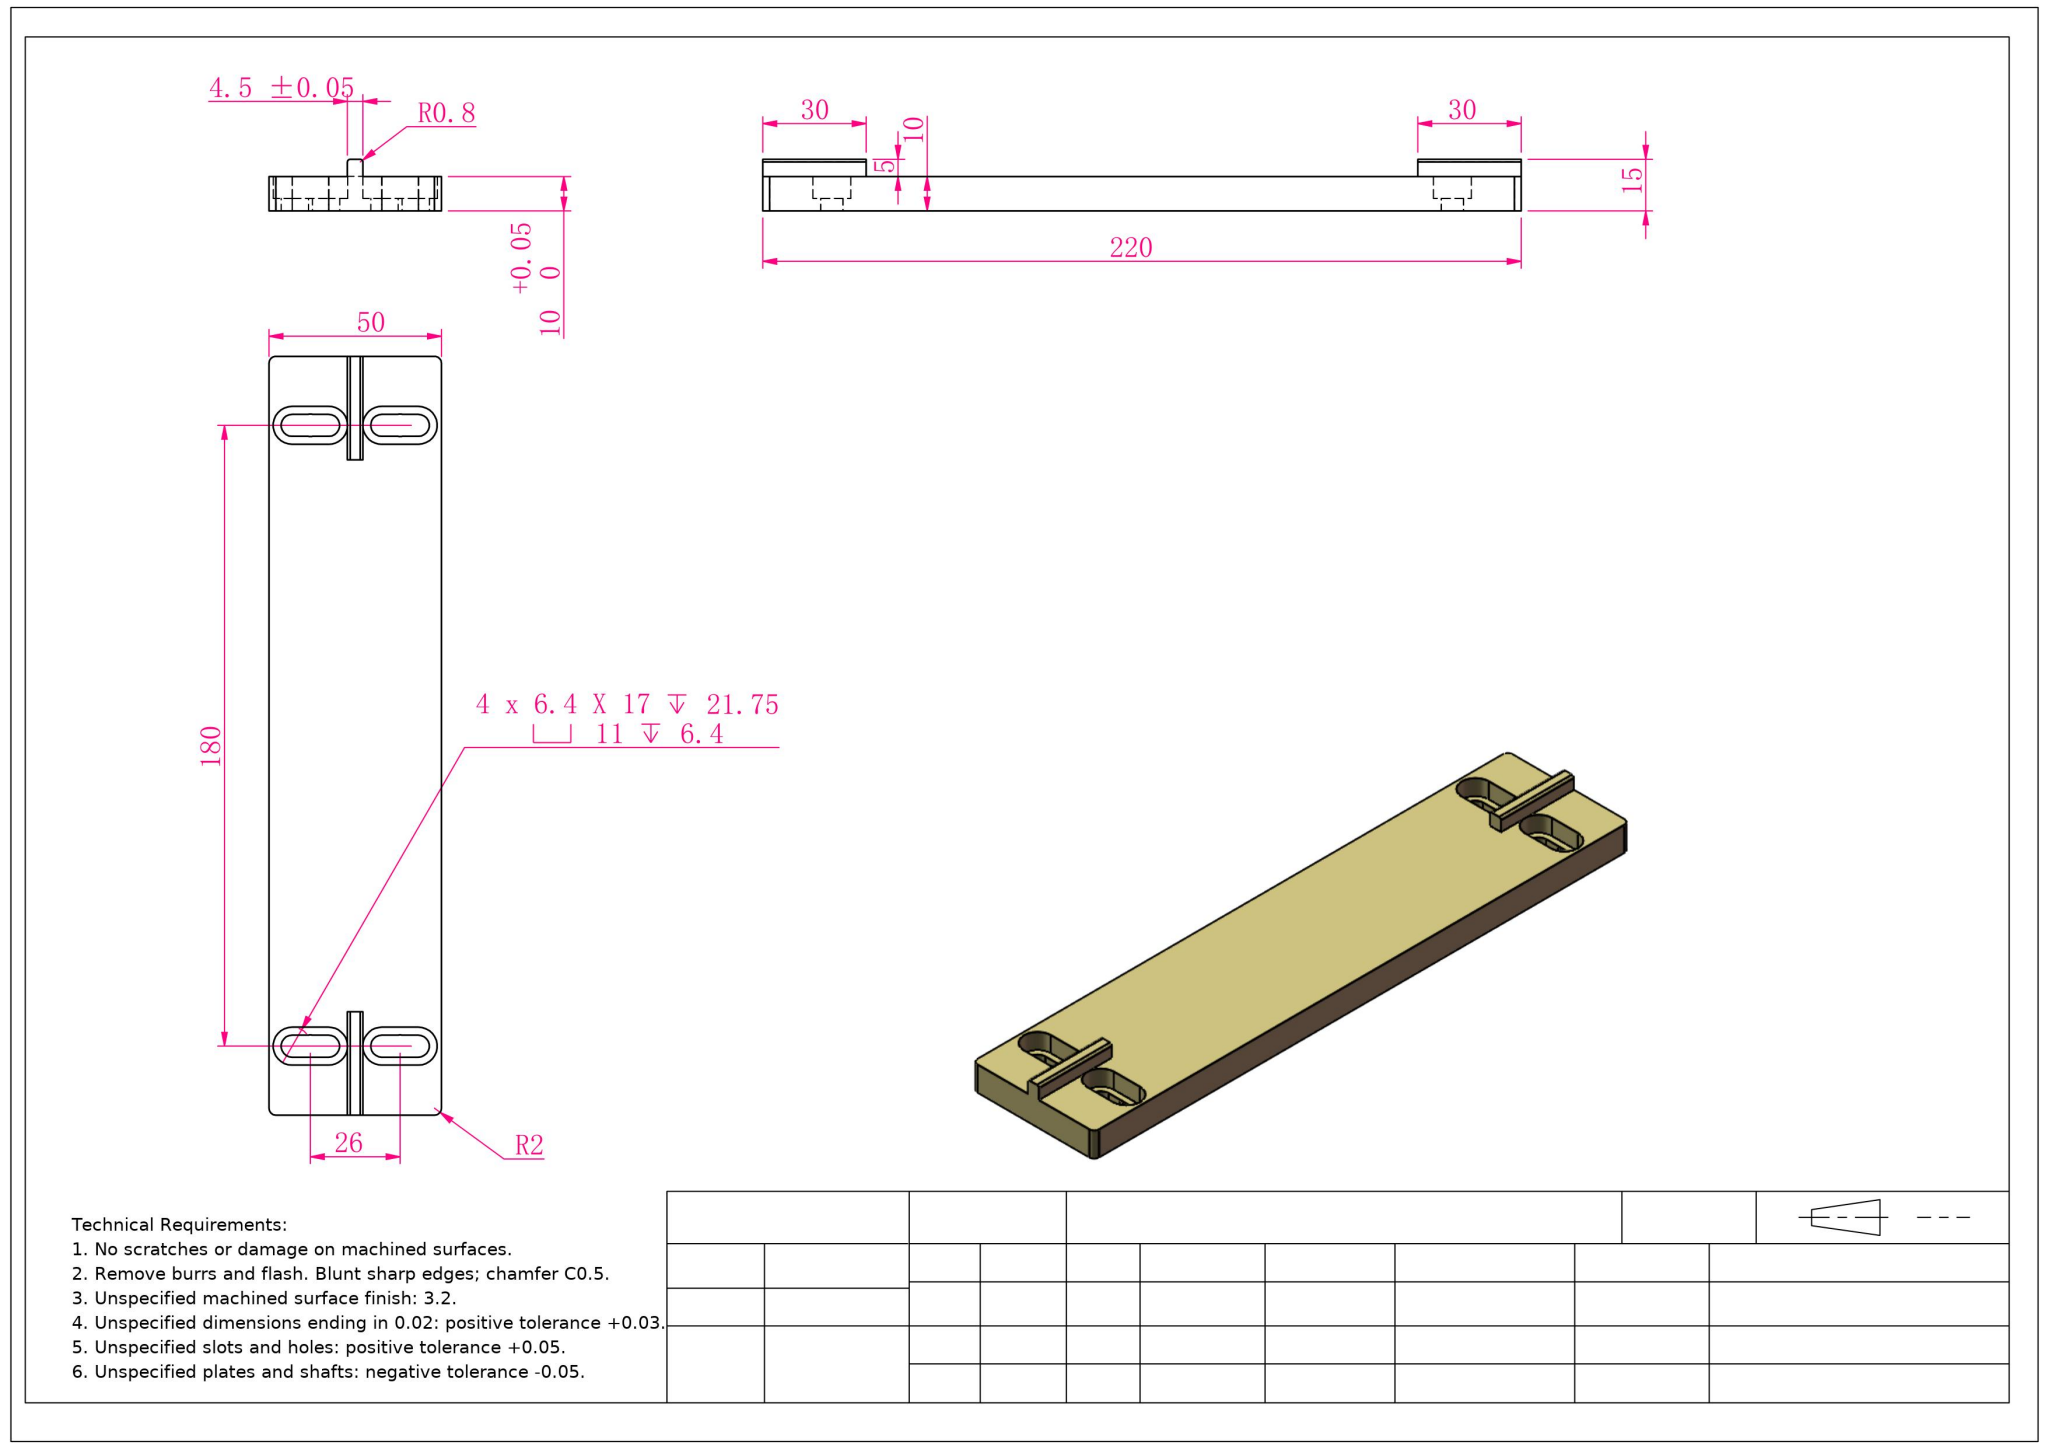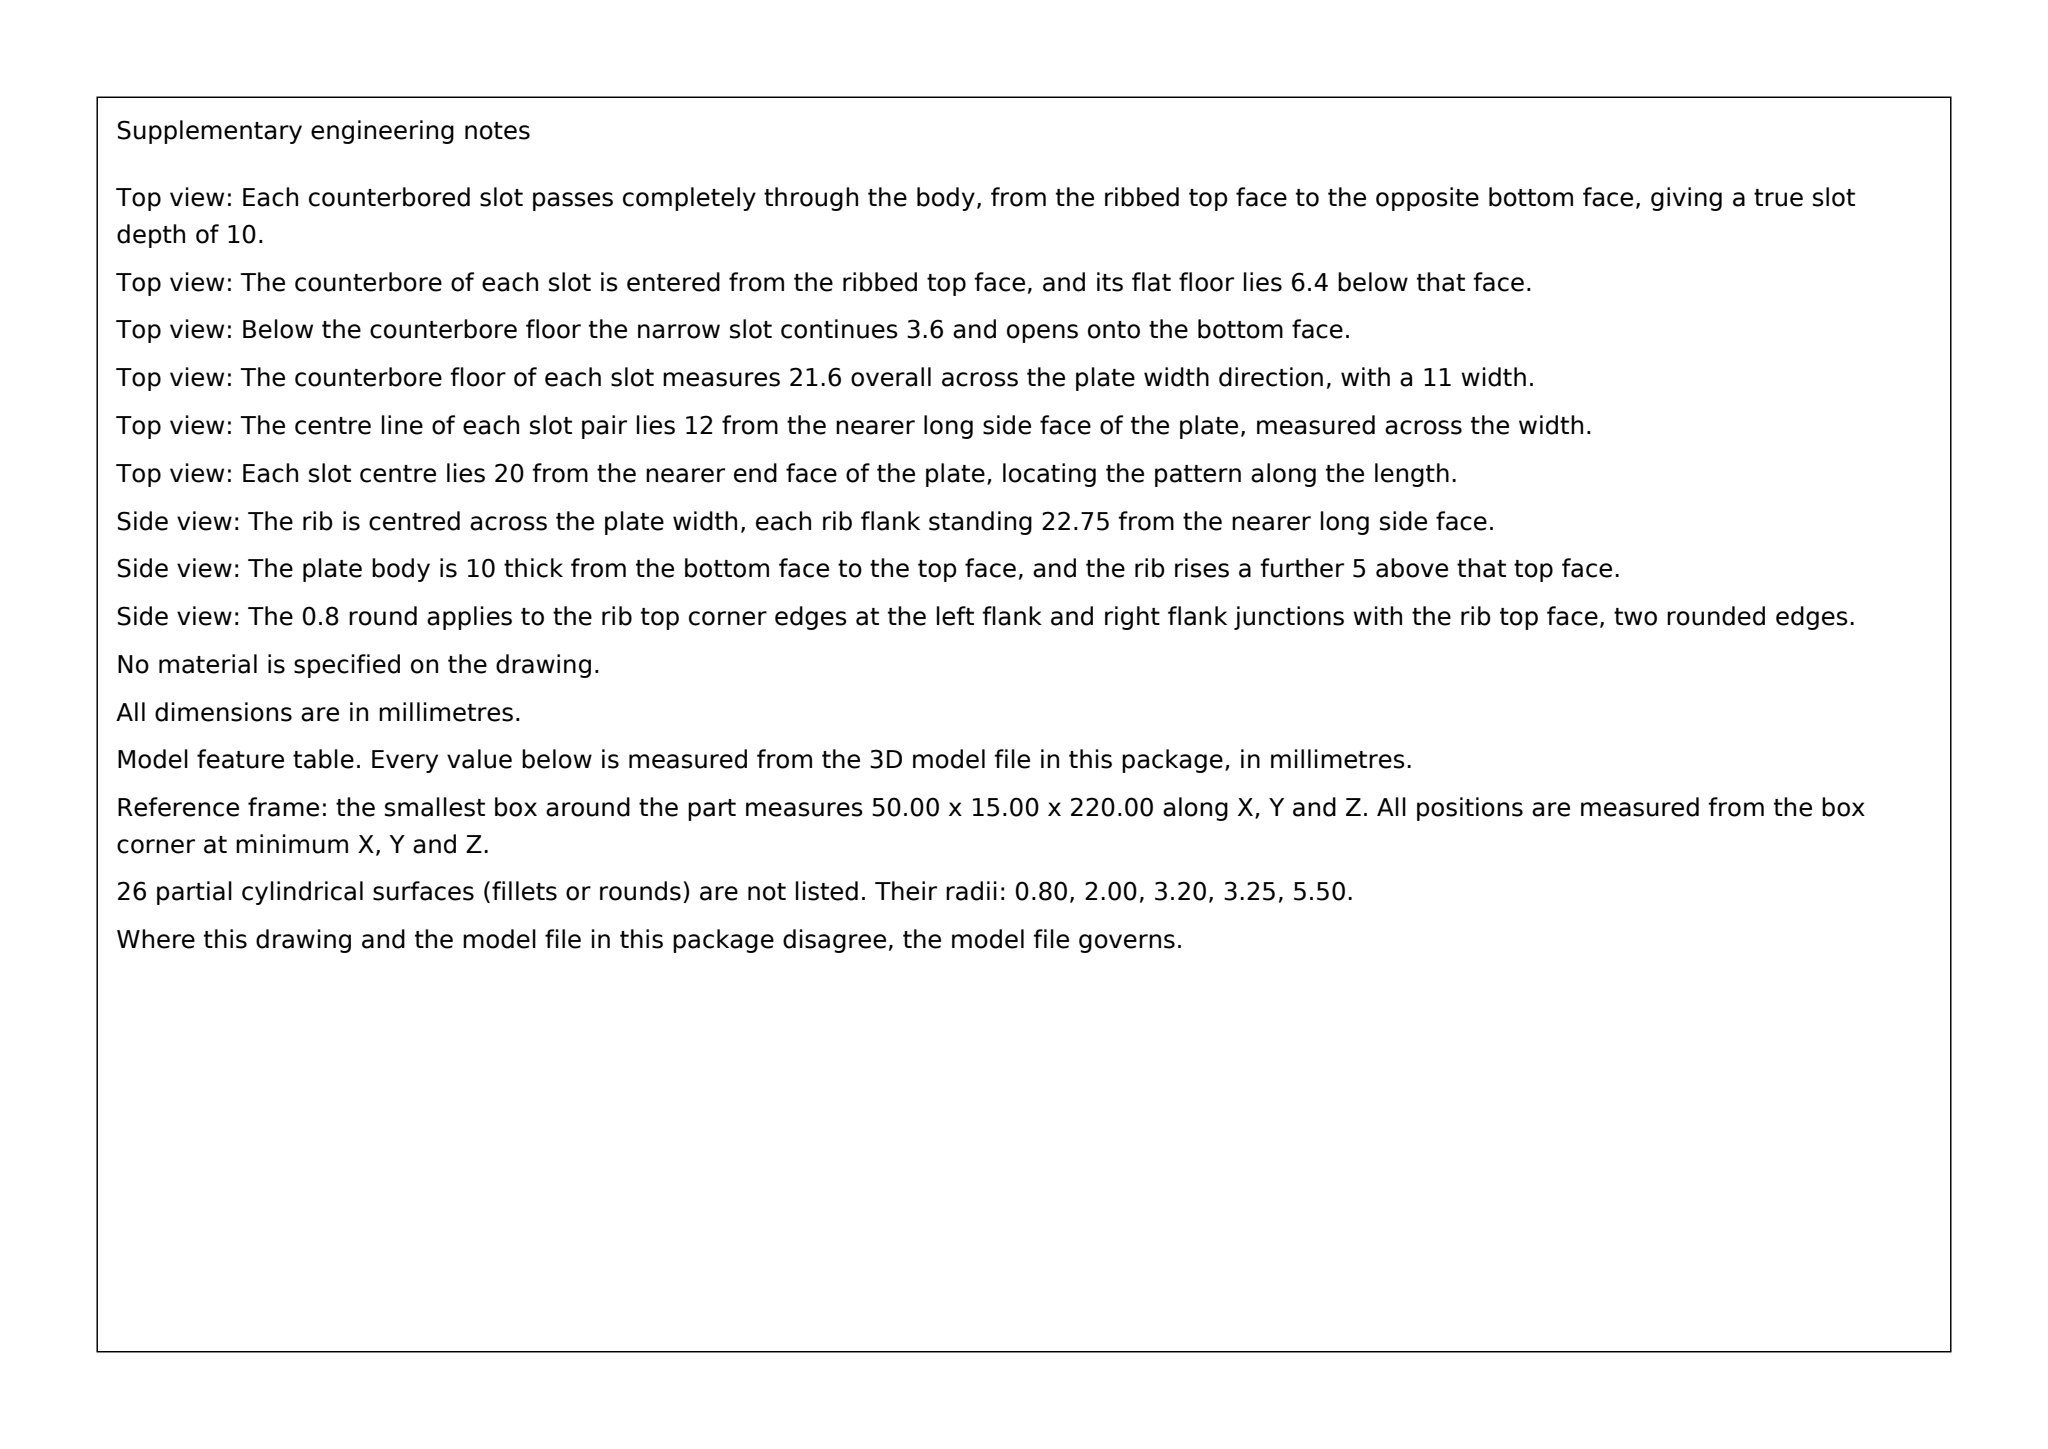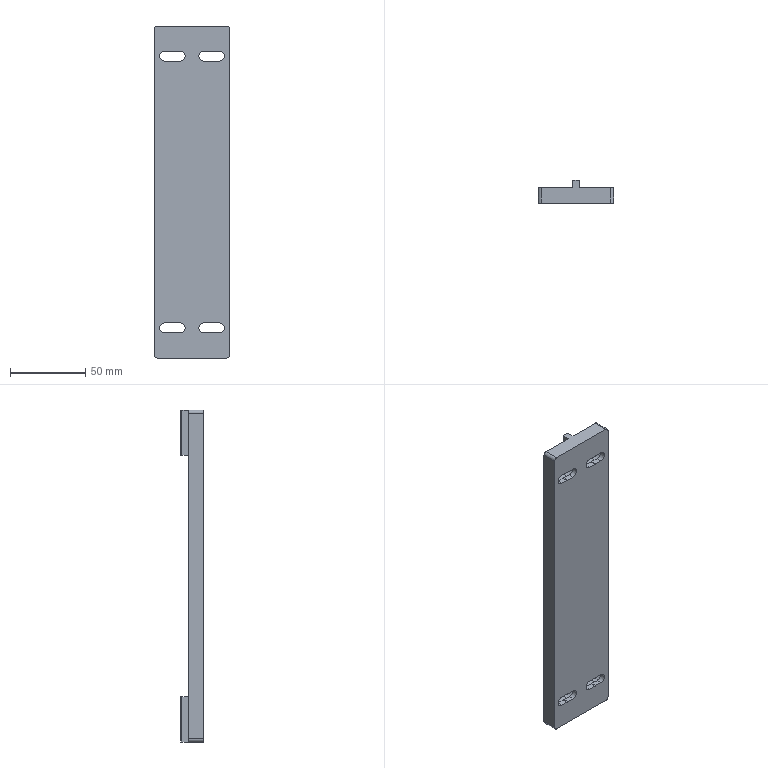Part | SolidWorks | mm | 1 solid | 78 faces | box 50 x 15 x 220 mm | volume 104440 mm3 | plane 46 | cylinder 32 | commonest cylinder face diameters 6.4 x8 11 x8 6.5 x8 1.6 x4 4 x4
Drawing notes:
TOP VIEW: SLOT CL 20 FROM END FACE (TYP BOTH ENDS) | from the solid: Slot arcs (Ø6.4/Ø11) axes at z=20.0 and z=200.0; part length z=0..220 (220-200=20)
TOP VIEW: 4.5 RIB CL 25 FROM SIDE EDGE (CTRD ON 50) | from the solid: Rib faces x=22.8 & 27.2 (R0.8 arcs at x=23.6/26.5, top y=15) -> CL x=25.0 of 50 wide
TOP VIEW: SLOT CL 12 FROM SIDE EDGE, 26 BETWEEN SLOT CL | from the solid: Slot mid arcs at x=12.0 and x=38.0; side faces x=0 and x=50 -> 12 and 26 spacing